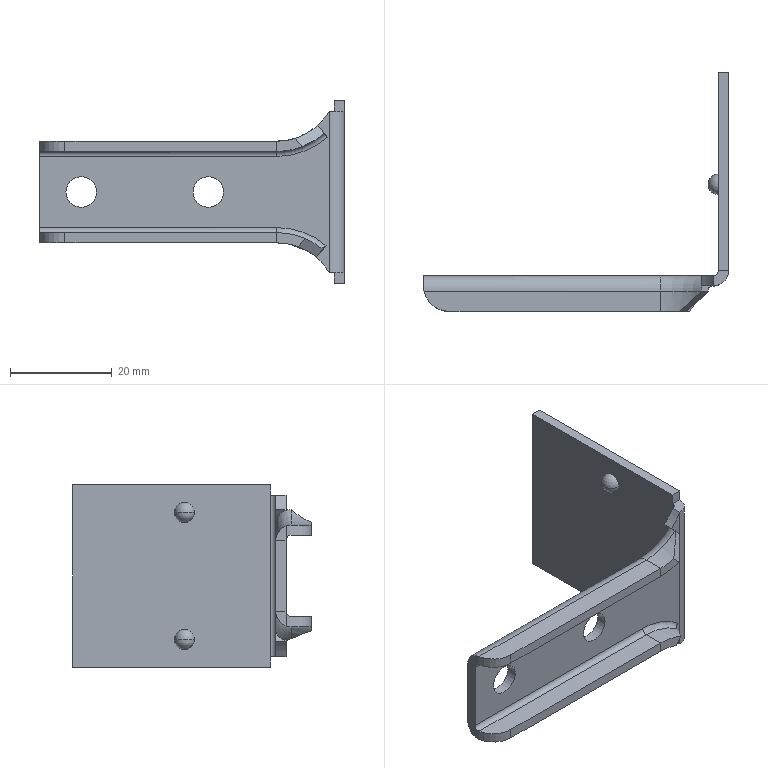Component | SolidWorks | Hinge(No.46)-1 | 1 solid | 62 faces | volume 6124 mm3 | plane 28 | cylinder 18 | torus 8 | sphere 8 | commonest cylinder face diameters 6 x7 24 x4 2 x3 28 x2 10 x2 | material Plain Carbon Steel